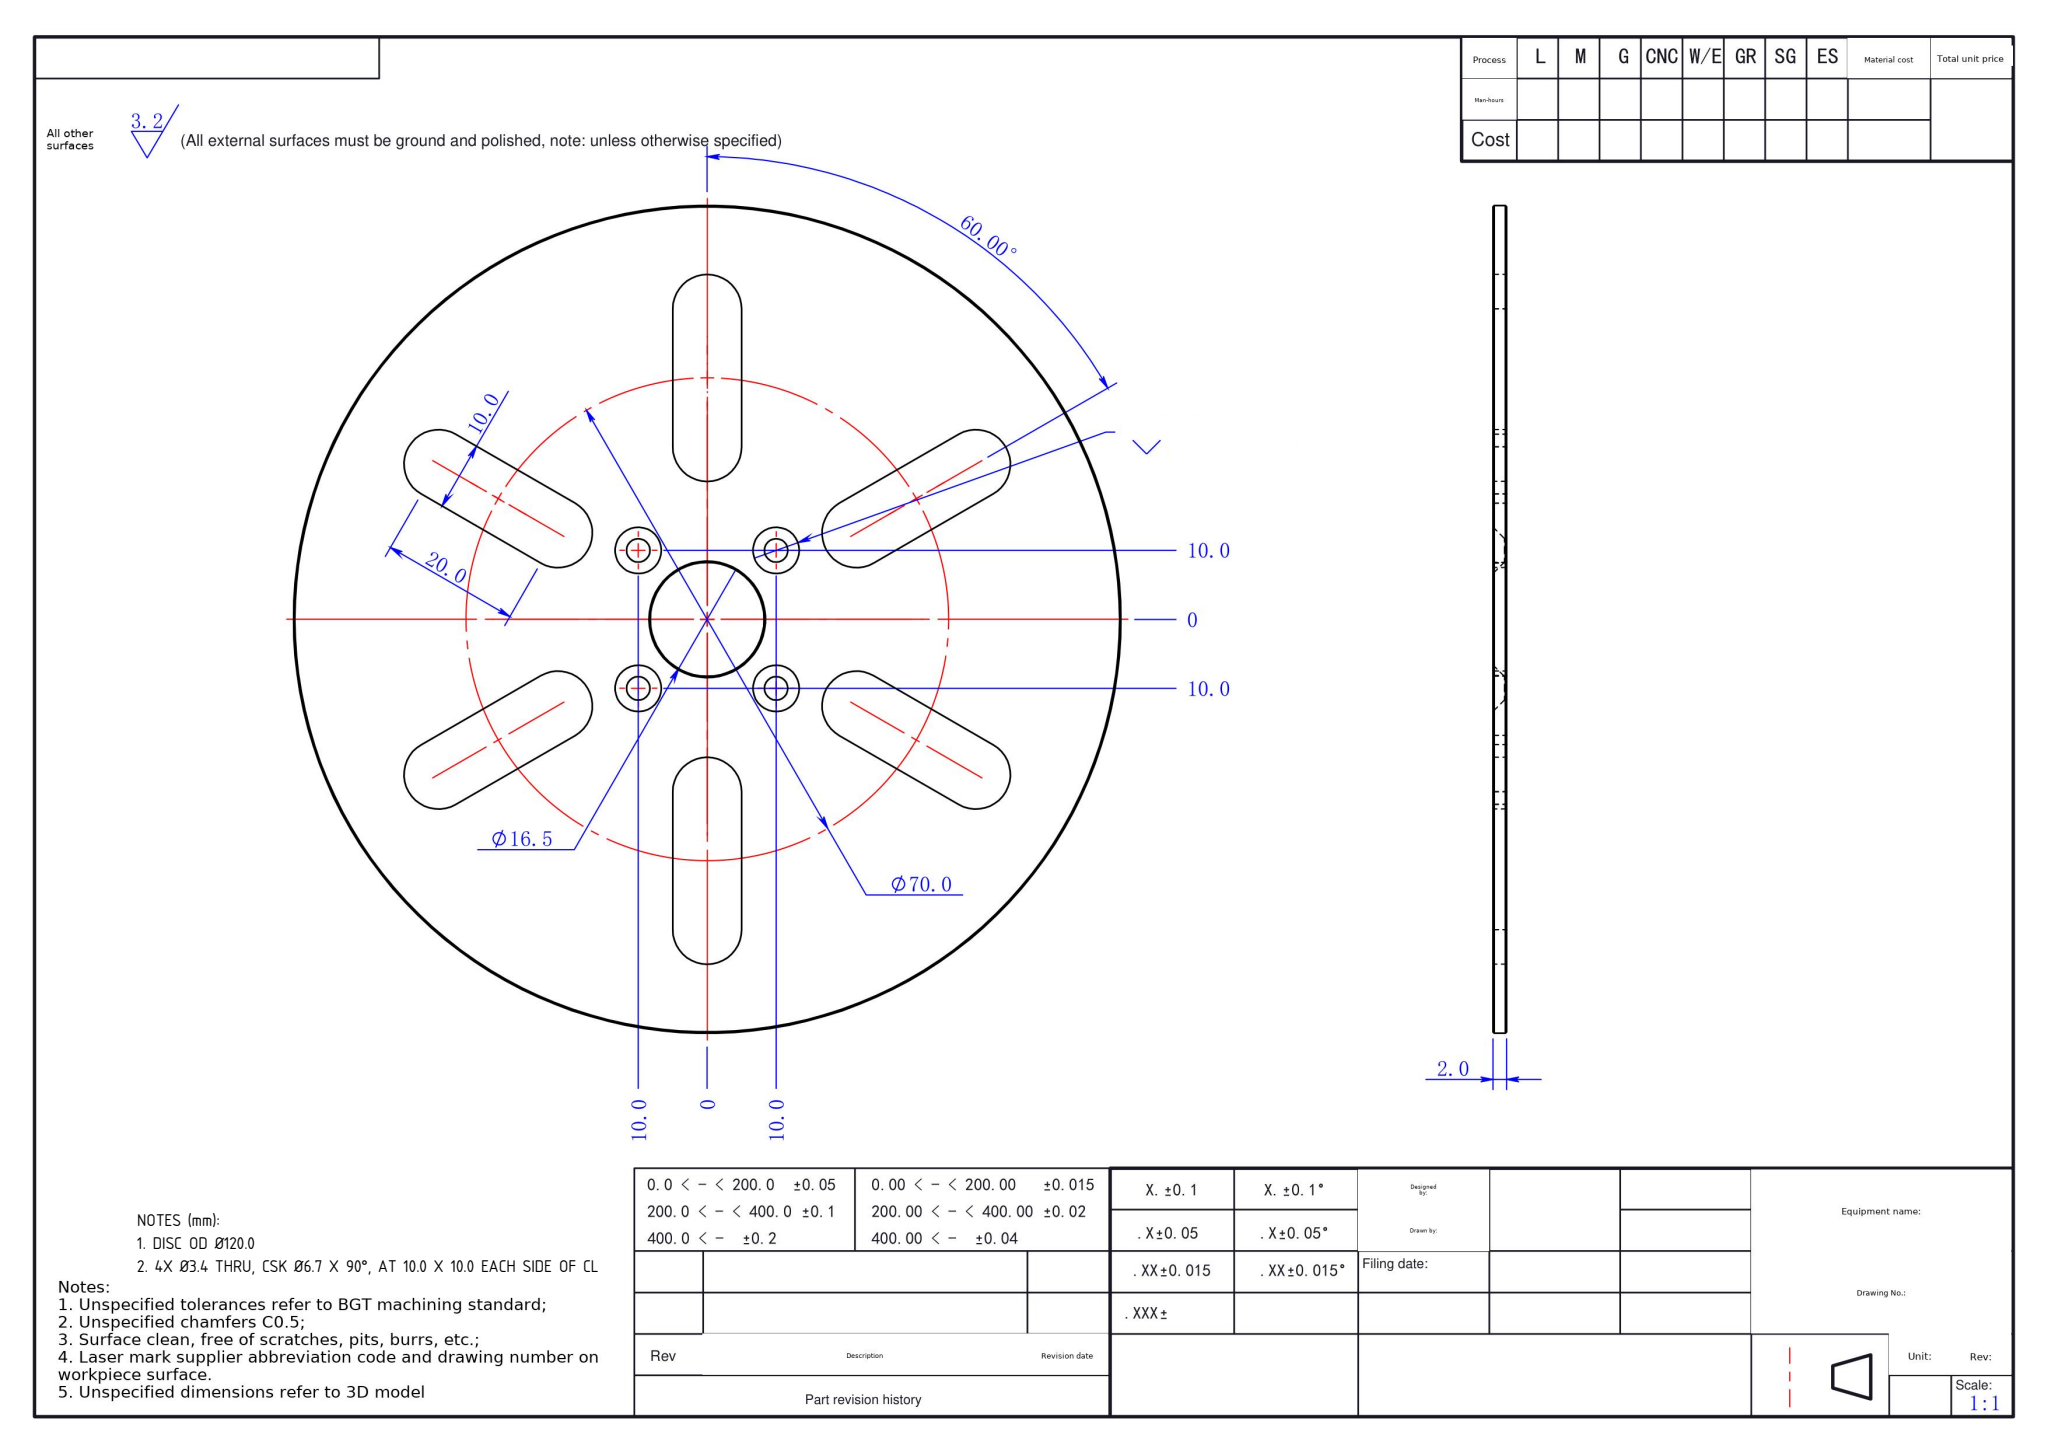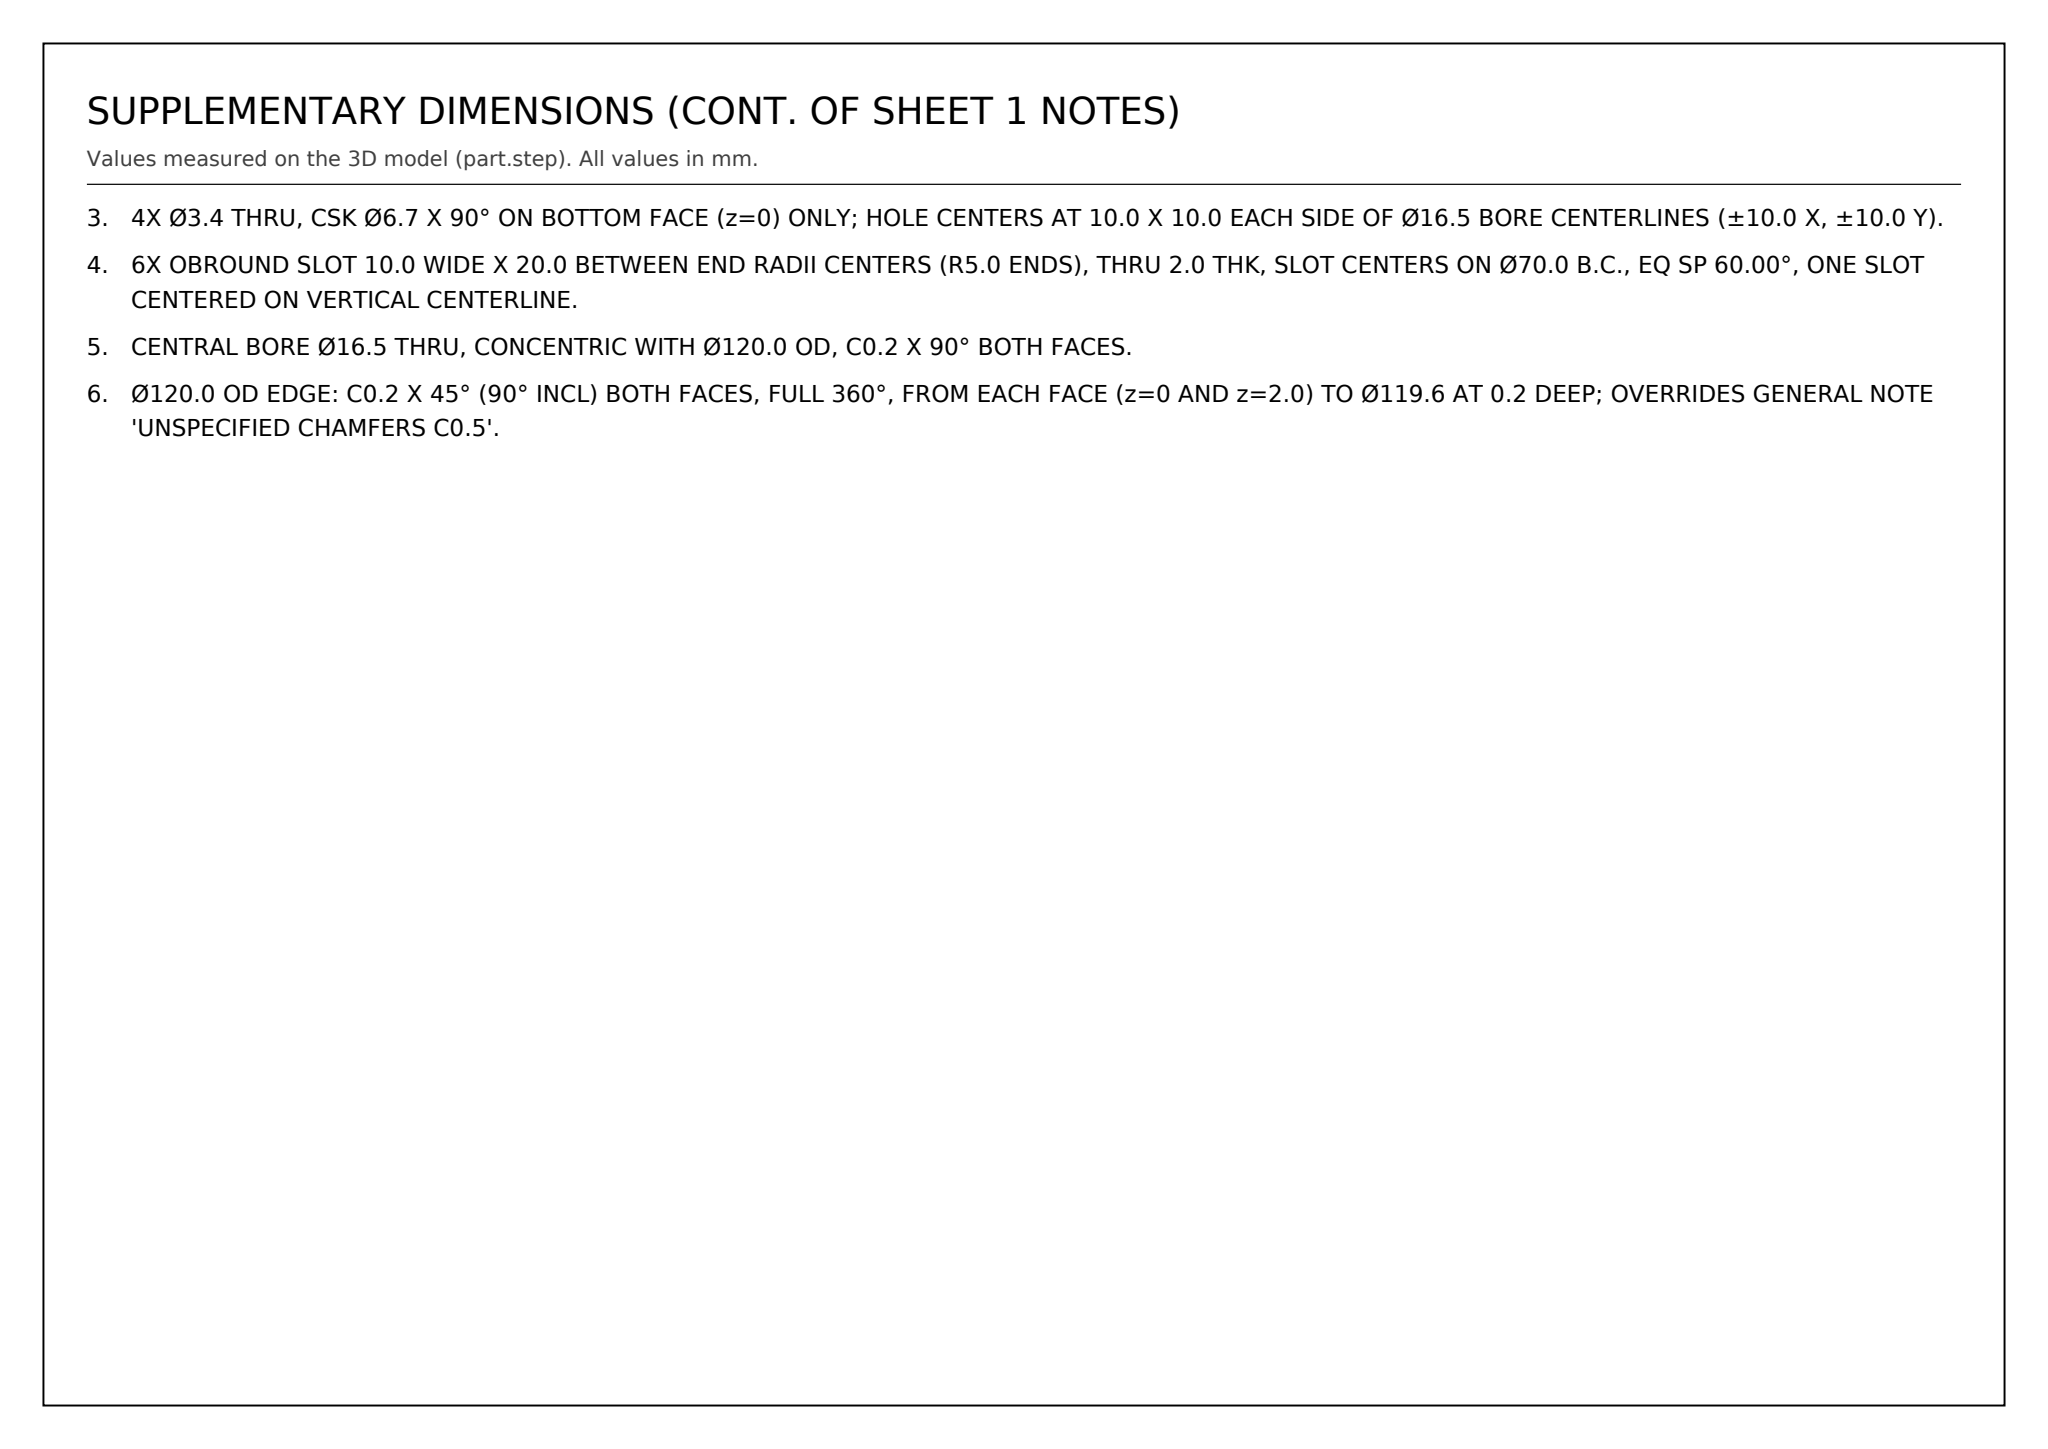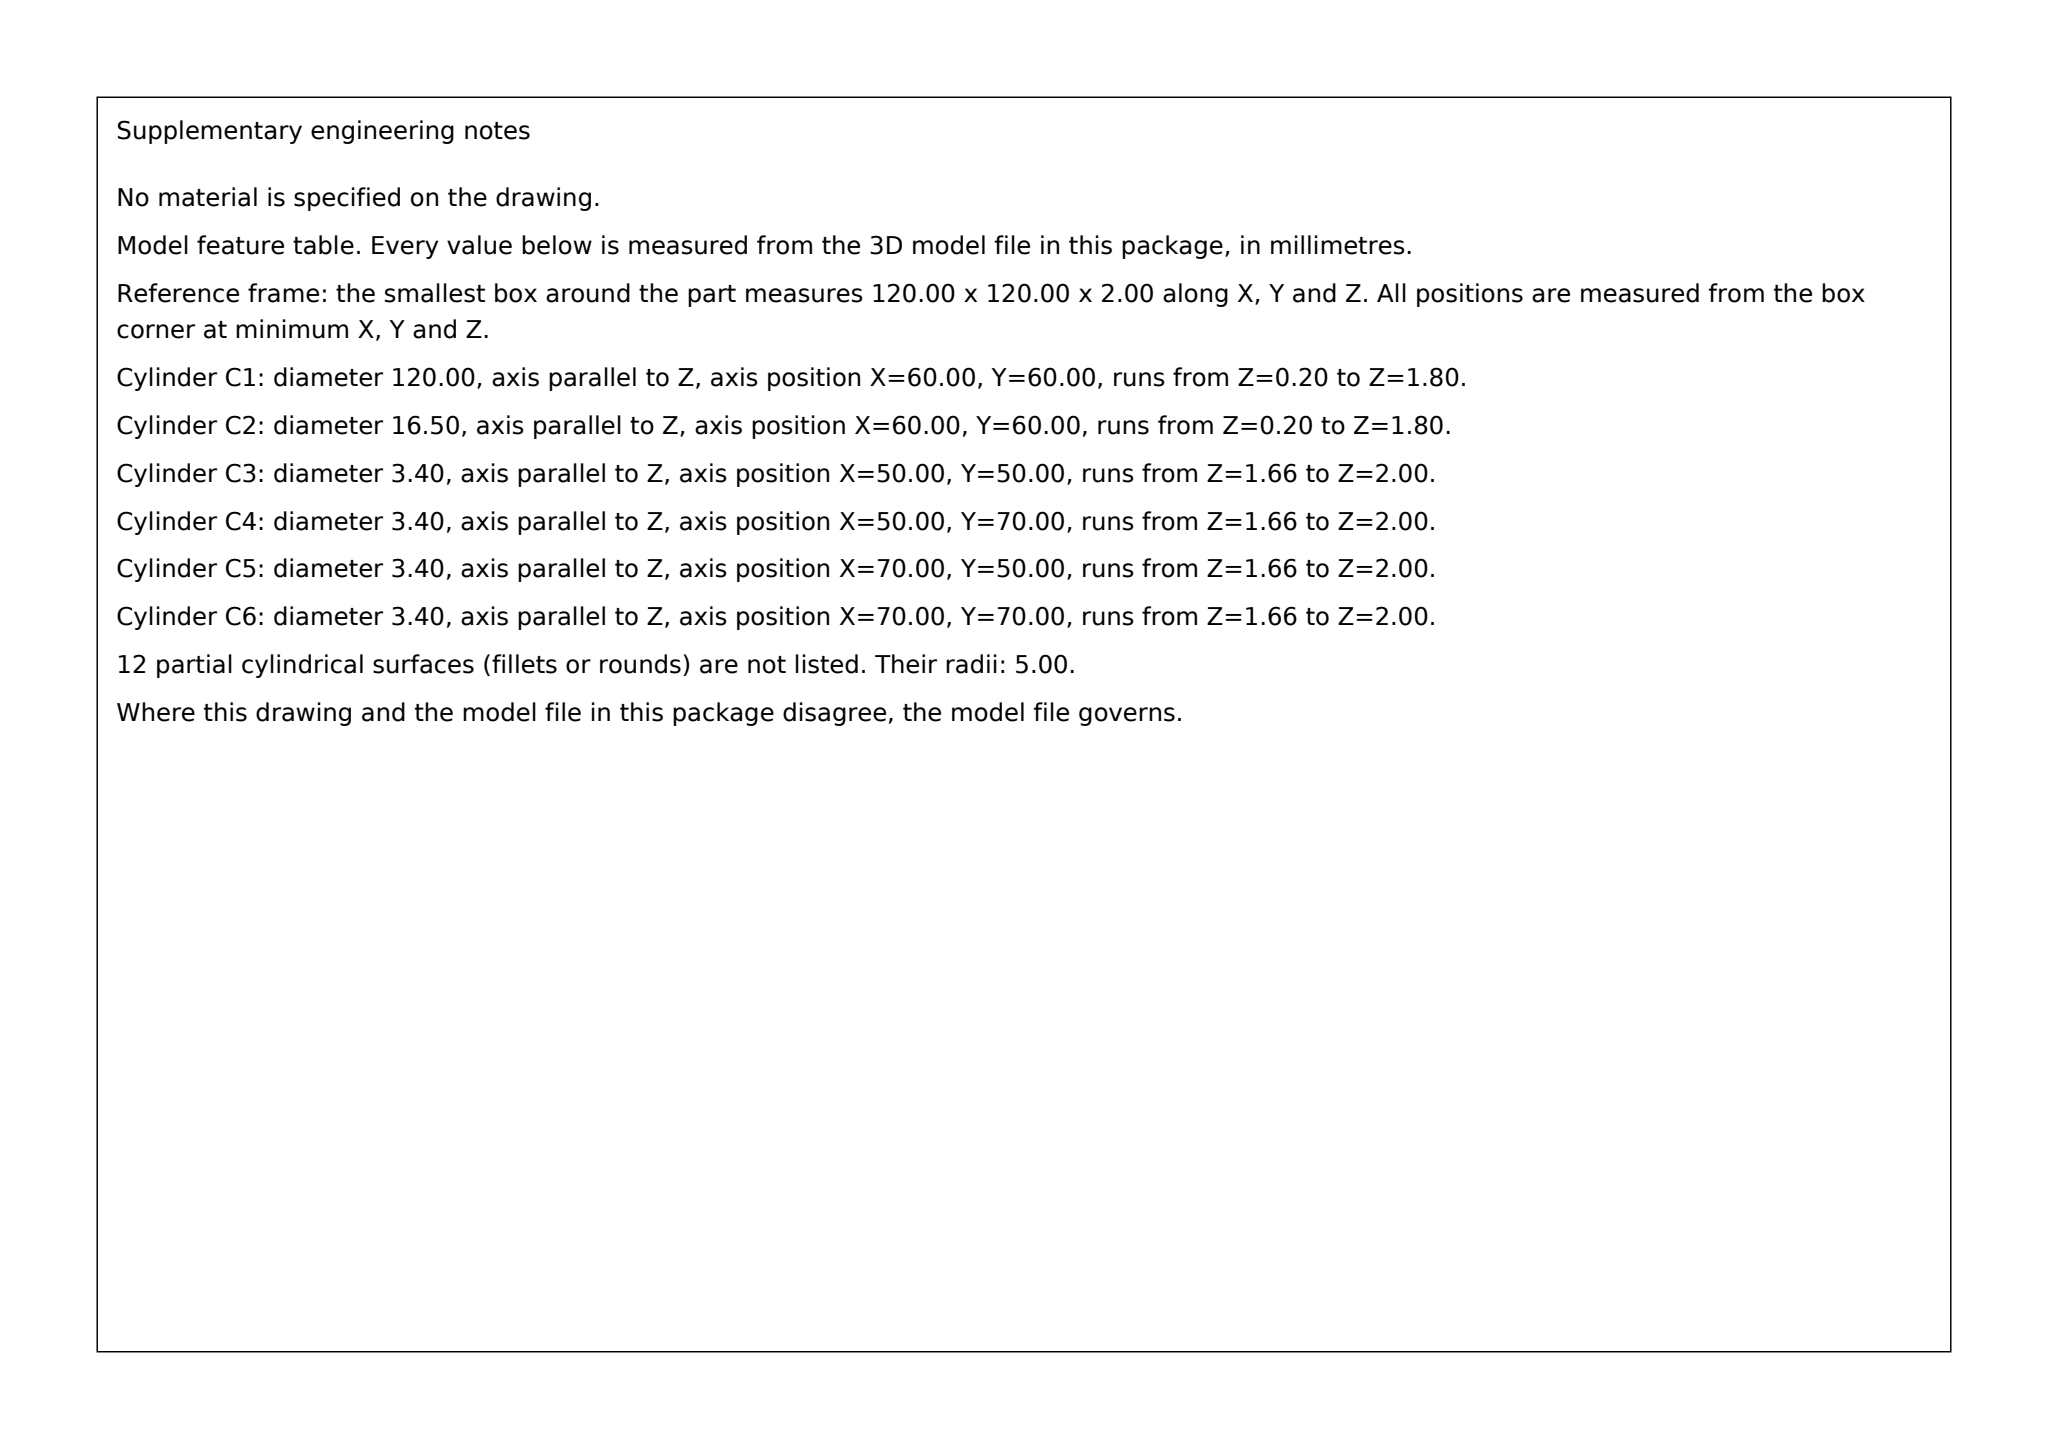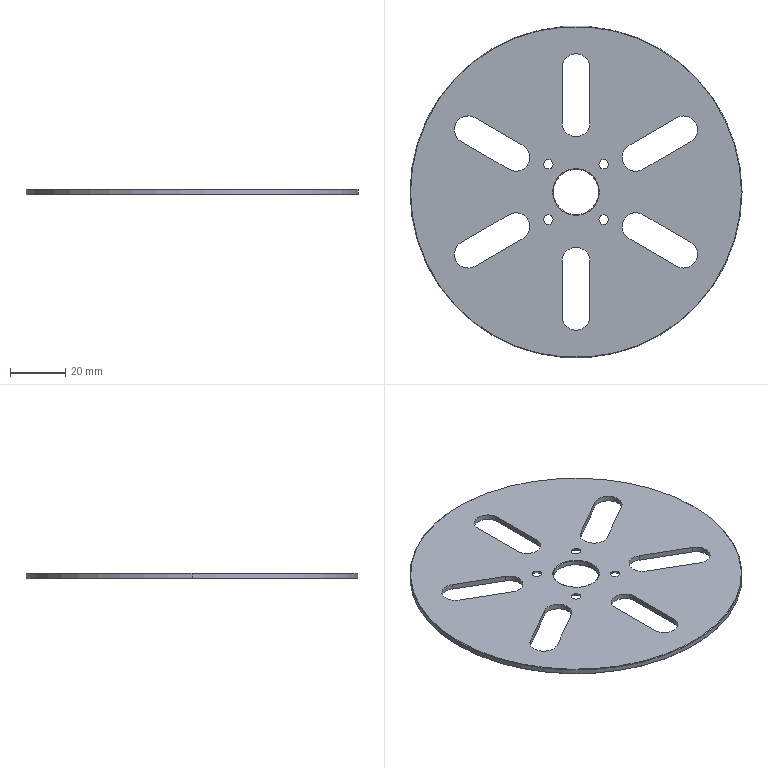Part | SolidWorks | mm | 1 solid | 58 faces | box 120 x 120 x 2 mm | volume 18682 mm3 | cylinder 28 | cone 16 | plane 14 | commonest cylinder face diameters 10 x16 3.4 x8 16.5 x2 120 x2
Drawing notes:
DISC OD Ø120.0 | from the solid: cylinder dia 120.0 axis z at [60.0,60.0], bbox 120x120x2.0
4X Ø3.4 THRU, CSK Ø6.7 X 90°, AT 10.0 X 10.0 EACH SIDE OF CL | from the solid: Ø3.4 z-cyls only at (50,50),(50,70),(70,50),(70,70) vs center (60,60); 90° csk ref dia 6.72
4X Ø3.4 THRU, CSK Ø6.7 X 90° ON BOTTOM FACE (z=0) ONLY; HOLE CENTERS AT 10.0 X 10.0 EACH SIDE OF Ø16.5 BORE CENTERLINES (±10.0 X, ±10.0 Y). | from the solid: cylinders hole/bore Ø3.4 (4 off) at (50,50),(50,70),(70,50),(70,70), z 1.7-2.0; cones 90° ref dia 6.72 starting at z=0.0, height 1.7
6X OBROUND SLOT 10.0 WIDE X 20.0 BETWEEN END RADII CENTERS (R5.0 ENDS), THRU 2.0 THK, SLOT CENTERS ON Ø70.0 B.C., EQ SP 60.00°, ONE SLOT CENTERED ON VERTICAL CENTERLINE. | from the solid: 12 concave Ø10.0 180° arcs (slot ends) paired at 35.0 radius from bore center (60,60); e.g. (60,85)&(60,105), (81.7,72.5)&(99,82.5); through z 0.0-2.0; flat faces x=55/65 extent y 15-35 and 85-105
CENTRAL BORE Ø16.5 THRU, CONCENTRIC WITH Ø120.0 OD, C0.2 X 90° BOTH FACES. | from the solid: cylinder hole/bore Ø16.5 at (60,60), z 0.2-1.8; cones 90° ref dia 16.5/16.9 at z=0.0 and z=1.8
Ø120.0 OD EDGE: C0.2 X 45° (90° INCL) BOTH FACES, FULL 360°, FROM EACH FACE (z=0 AND z=2.0) TO Ø119.6 AT 0.2 DEEP; OVERRIDES GENERAL NOTE 'UNSPECIFIED CHAMFERS C0.5'. | from the solid: cones[90.0, ref_dia 120.0, bbox_from z=0.0, size z 0.2] and cones[90.0, ref_dia 119.6, bbox_from z=1.8, size z 0.2]; OD cylinder Ø120.0 spans z 0.2 to 1.8 while faces at z=0 and z=2.0 extend to 119.8
build123d program:
from build123d import *

# Parameters (mm, degrees)
SKETCH1_R                                    = 60
SKETCH1_R_2                                  = 8.25
BOSS_EXTRUDE1_DEPTH                          = 2
M3_HEXAGON_SOCKET_COUNTERSUNK_HEAD_S_2_COUNT = 2
M3_HEXAGON_SOCKET_COUNTERSUNK_HEAD_S_2_PITCH = 14.142
M3_HEXAGON_SOCKET_COUNTERSUNK_HEAD_S_3_COUNT = 2
M3_HEXAGON_SOCKET_COUNTERSUNK_HEAD_S_3_PITCH = 28.284
M3_HEXAGON_SOCKET_COUNTERSUNK_HEAD_S_4_COUNT = 2
M3_HEXAGON_SOCKET_COUNTERSUNK_HEAD_S_4_PITCH = 20
M3_HEXAGON_SOCKET_COUNTERSUNK_HEAD_S_5_COUNT = 2
M3_HEXAGON_SOCKET_COUNTERSUNK_HEAD_S_5_PITCH = 20
CUT_EXTRUDE1_DEPTH                           = 85.876
CIRPATTERN1_COUNT                            = 6
CHAMFER1_SIZE                                = 0.2


with BuildPart() as part:
    # Sketch1 → Boss-Extrude1 (new body)
    with BuildSketch(Plane.XY):
        Circle(SKETCH1_R)
        Circle(SKETCH1_R_2, mode=Mode.SUBTRACT)
    extrude(amount=BOSS_EXTRUDE1_DEPTH)

    # Sketch3 → M3 Hexagon Socket Countersunk Head Screw (revolve, cut)
    with BuildSketch(Plane(origin=(-10, 10, 0), x_dir=(0, 1, 0), z_dir=(1, 0, 0))):
        Polygon((0, 0), (0, 2), (1.7, 2), (1.7, 1.66), (3.36, 0), align=None)
    m3_hexagon_socket_countersunk_head_screw = revolve(axis=Axis((-10, 10, -6.35), (0, 0, 1)), mode=Mode.SUBTRACT)

    # M3 Hexagon Socket Countersunk Head S 2: M3 Hexagon Socket Countersunk Head Screw ×2
    with Locations(*[Vector(0.7071, -0.7071, 0) * (i * M3_HEXAGON_SOCKET_COUNTERSUNK_HEAD_S_2_PITCH) for i in range(1, M3_HEXAGON_SOCKET_COUNTERSUNK_HEAD_S_2_COUNT)]):
        add(m3_hexagon_socket_countersunk_head_screw, mode=Mode.SUBTRACT)

    # M3 Hexagon Socket Countersunk Head S 3: M3 Hexagon Socket Countersunk Head Screw ×2
    with Locations(*[Vector(0.7071, -0.7071, 0) * (i * M3_HEXAGON_SOCKET_COUNTERSUNK_HEAD_S_3_PITCH) for i in range(1, M3_HEXAGON_SOCKET_COUNTERSUNK_HEAD_S_3_COUNT)]):
        add(m3_hexagon_socket_countersunk_head_screw, mode=Mode.SUBTRACT)

    # M3 Hexagon Socket Countersunk Head S 4: M3 Hexagon Socket Countersunk Head Screw ×2
    with Locations(*[(0, -i * M3_HEXAGON_SOCKET_COUNTERSUNK_HEAD_S_4_PITCH, 0) for i in range(1, M3_HEXAGON_SOCKET_COUNTERSUNK_HEAD_S_4_COUNT)]):
        add(m3_hexagon_socket_countersunk_head_screw, mode=Mode.SUBTRACT)

    # M3 Hexagon Socket Countersunk Head S 5: M3 Hexagon Socket Countersunk Head Screw ×2
    with Locations(*[(i * M3_HEXAGON_SOCKET_COUNTERSUNK_HEAD_S_5_PITCH, 0, 0) for i in range(1, M3_HEXAGON_SOCKET_COUNTERSUNK_HEAD_S_5_COUNT)]):
        add(m3_hexagon_socket_countersunk_head_screw, mode=Mode.SUBTRACT)

    # Sketch4 → Cut-Extrude1 (cut, through all)
    with BuildSketch(Plane(origin=(0, 0, 0), x_dir=(-1, 0, 0), z_dir=(0, 0, -1))):
        with BuildLine():
            Line((-5, 25), (-5, 45))
            ThreePointArc((-5, 45), (0, 50), (5, 45))
            Line((5, 45), (5, 25))
            ThreePointArc((5, 25), (0, 20), (-5, 25))
        make_face()
    cut_extrude1 = extrude(amount=-CUT_EXTRUDE1_DEPTH, mode=Mode.SUBTRACT)

    # CirPattern1: Cut-Extrude1 ×6 about axis
    cirpattern1_axis = Axis((0, 0, 0), (0, 0, 1))
    for i in range(1, CIRPATTERN1_COUNT):
        add(cut_extrude1.rotate(cirpattern1_axis, i * 360 / CIRPATTERN1_COUNT), mode=Mode.SUBTRACT)

    # Chamfer1
    chamfer1_edges = [part.edges().sort_by_distance(p)[0] for p in [
        (-60, 0, 0),
        (-60, 0, 2),
        (-8.25, 0, 0),
        (-8.25, 0, 2),
    ]]
    chamfer(chamfer1_edges, length=CHAMFER1_SIZE)


solid = part.part